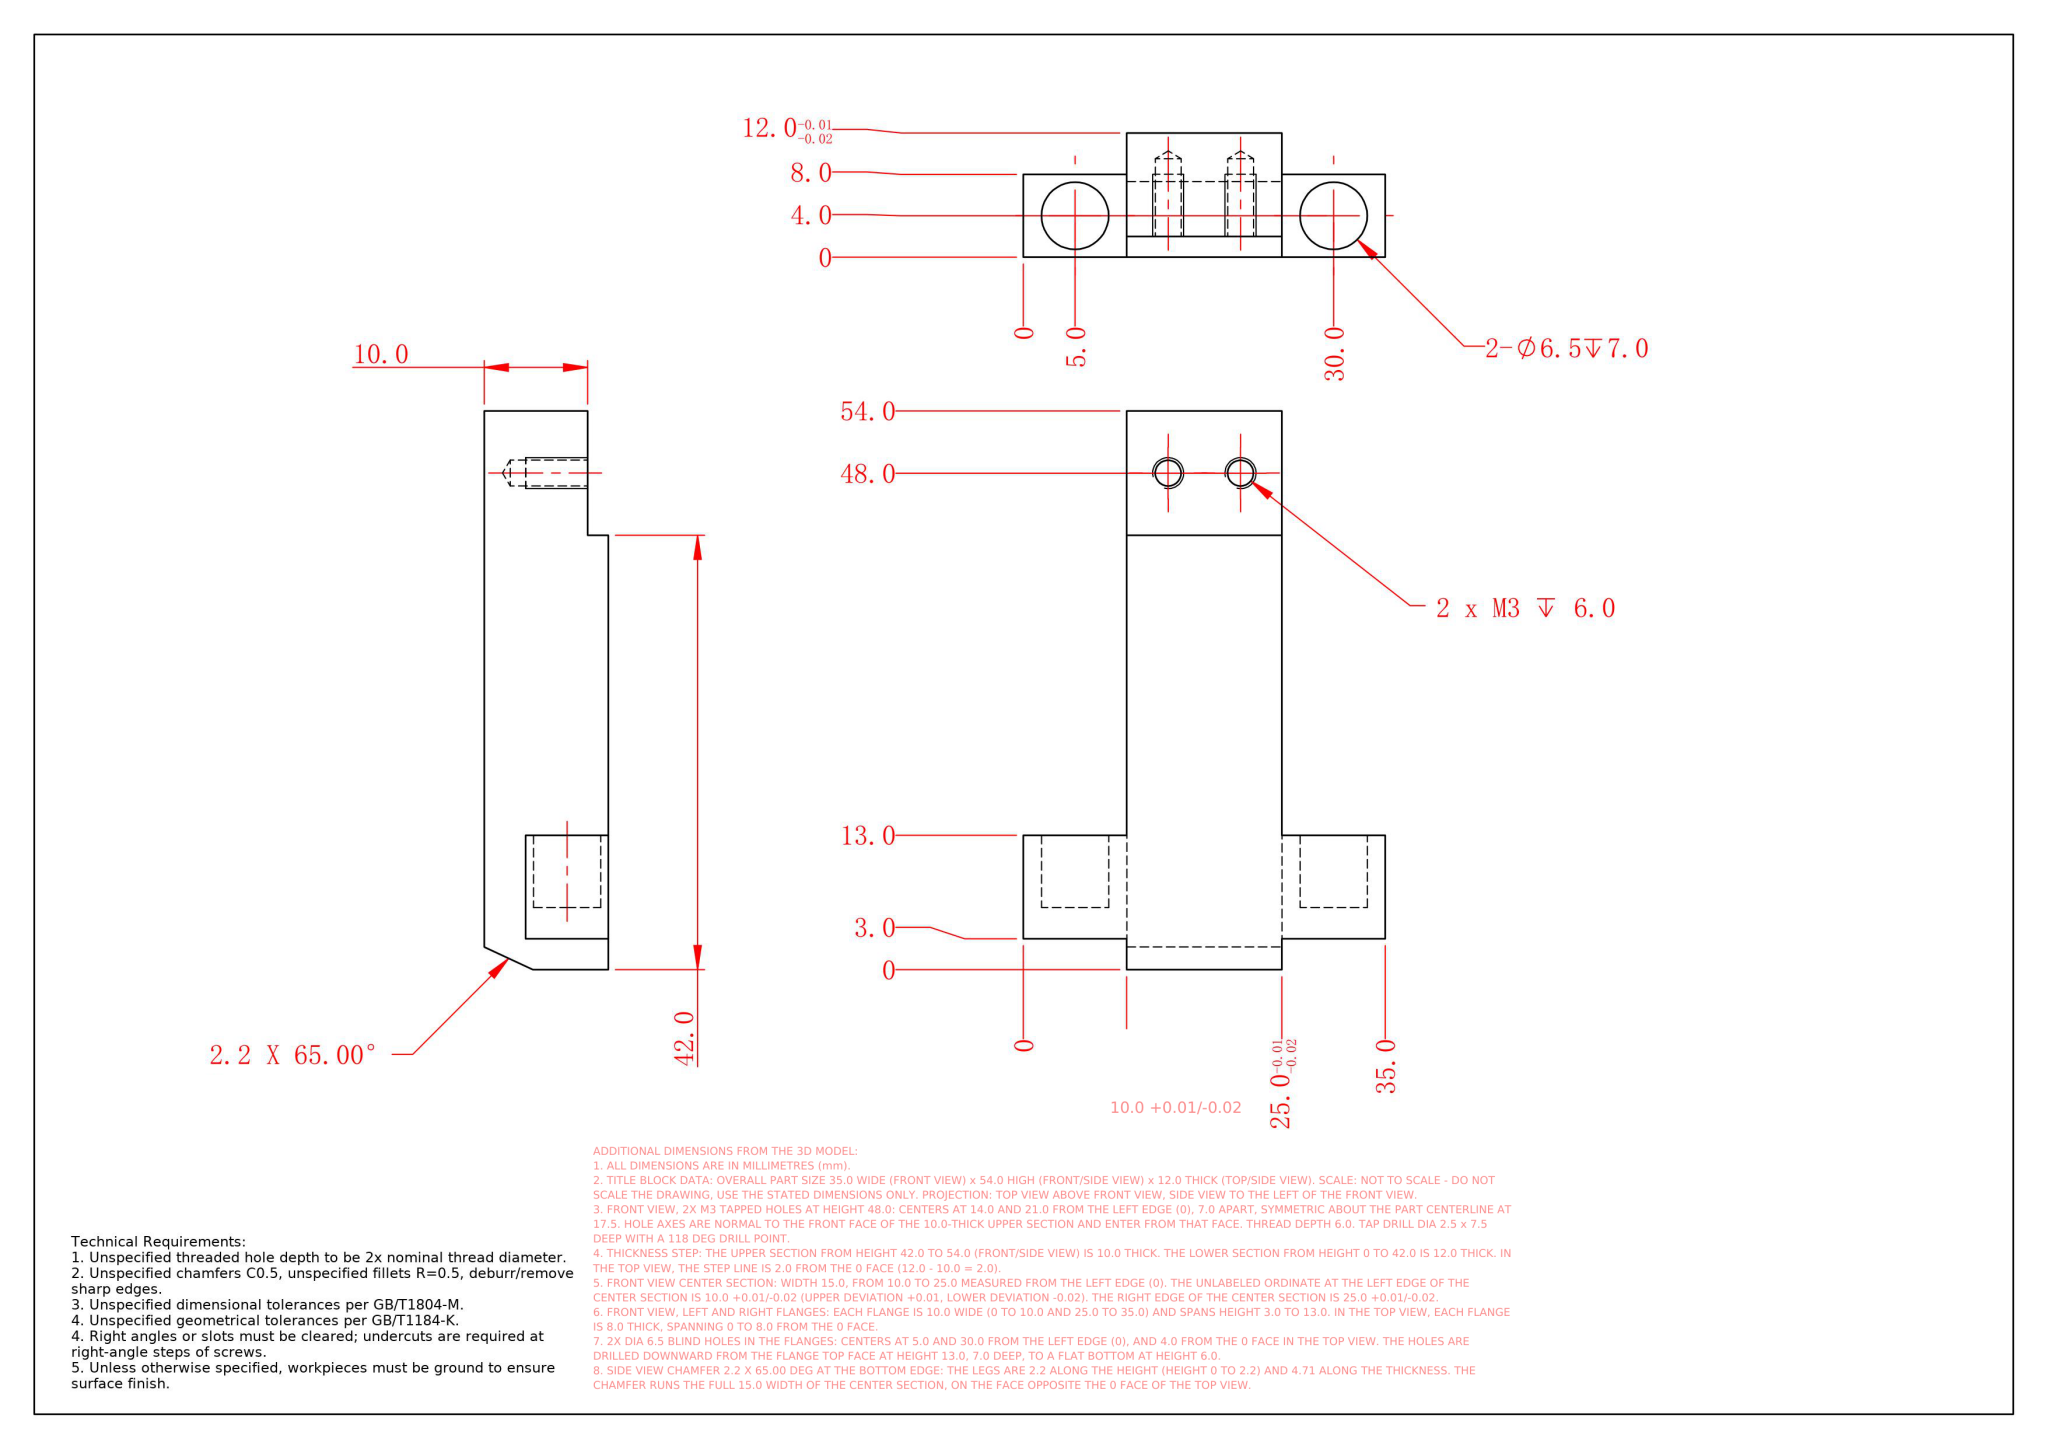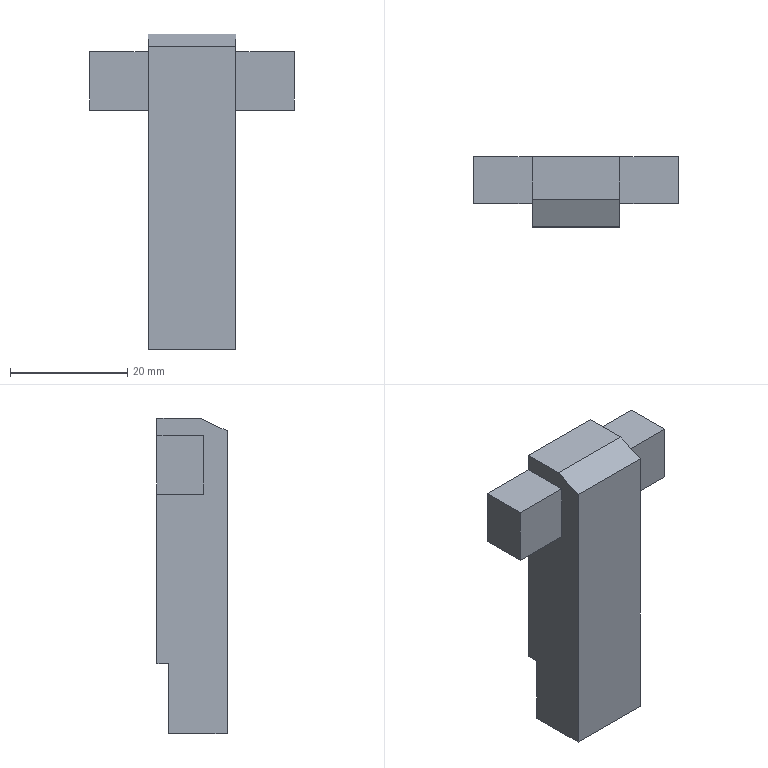Part | NX | mm | 1 solid | 31 faces | box 35 x 12 x 54 mm | volume 10342 mm3 | plane 19 | cylinder 8 | cone 4 | commonest cylinder face diameters 2.5 x4 6.5 x4
STEP:
#1=COLOUR_RGB('',0.7529,0.7529,0.7529);
#2=FILL_AREA_STYLE_COLOUR('',#1);
#3=FILL_AREA_STYLE('',(#2));
#4=SURFACE_STYLE_FILL_AREA(#3);
#5=SURFACE_SIDE_STYLE('',(#4));
#6=SURFACE_STYLE_USAGE(.BOTH.,#5);
#7=PRESENTATION_STYLE_ASSIGNMENT((#6));
#8=CARTESIAN_POINT('',(3.5,2.5,-23.25));
#9=VERTEX_POINT('',#8);
#10=CARTESIAN_POINT('',(3.5,2.5,-20.75));
#11=VERTEX_POINT('',#10);
#12=CARTESIAN_POINT('',(3.5,2.5,-22.));
#13=DIRECTION('',(0.,1.,0.));
#14=DIRECTION('',(0.,0.,1.));
#15=AXIS2_PLACEMENT_3D('',#12,#13,#14);
#16=CIRCLE('',#15,1.25);
#17=EDGE_CURVE('',#9,#11,#16,.T.);
#18=ORIENTED_EDGE('',*,*,#17,.F.);
#19=CARTESIAN_POINT('',(3.5,10.,-23.25));
#20=VERTEX_POINT('',#19);
#21=CARTESIAN_POINT('',(3.5,10.,-23.25));
#22=DIRECTION('',(0.,1.,0.));
#23=VECTOR('',#22,1000.);
#24=LINE('',#21,#23);
#25=EDGE_CURVE('',#9,#20,#24,.T.);
#26=ORIENTED_EDGE('',*,*,#25,.T.);
#27=CARTESIAN_POINT('',(3.5,10.,-20.75));
#28=VERTEX_POINT('',#27);
#29=CARTESIAN_POINT('',(3.5,10.,-22.));
#30=DIRECTION('',(0.,1.,0.));
#31=DIRECTION('',(0.,0.,1.));
#32=AXIS2_PLACEMENT_3D('',#29,#30,#31);
#33=CIRCLE('',#32,1.25);
#34=EDGE_CURVE('',#20,#28,#33,.T.);
#35=ORIENTED_EDGE('',*,*,#34,.T.);
#36=CARTESIAN_POINT('',(3.5,10.,-20.75));
#37=DIRECTION('',(0.,1.,0.));
#38=VECTOR('',#37,1000.);
#39=LINE('',#36,#38);
#40=EDGE_CURVE('',#11,#28,#39,.T.);
#41=ORIENTED_EDGE('',*,*,#40,.F.);
#42=EDGE_LOOP('',(#18,#26,#35,#41));
#43=FACE_OUTER_BOUND('',#42,.T.);
#44=CARTESIAN_POINT('',(3.5,10.,-22.));
#45=DIRECTION('',(0.,1.,0.));
#46=DIRECTION('',(0.,0.,1.));
#47=AXIS2_PLACEMENT_3D('',#44,#45,#46);
#48=CYLINDRICAL_SURFACE('',#47,1.25);
#49=ADVANCED_FACE('',(#43),#48,.F.);
#50=STYLED_ITEM('',(#7),#49);
#51=PRESENTATION_LAYER_ASSIGNMENT('','',(#50));
#52=COLOUR_RGB('',0.7529,0.7529,0.7529);
#53=FILL_AREA_STYLE_COLOUR('',#52);
#54=FILL_AREA_STYLE('',(#53));
#55=SURFACE_STYLE_FILL_AREA(#54);
#56=SURFACE_SIDE_STYLE('',(#55));
#57=SURFACE_STYLE_USAGE(.BOTH.,#56);
#58=PRESENTATION_STYLE_ASSIGNMENT((#57));
#59=ORIENTED_EDGE('',*,*,#25,.F.);
#60=CARTESIAN_POINT('',(3.5,2.5,-22.));
#61=DIRECTION('',(0.,1.,0.));
#62=DIRECTION('',(0.,0.,1.));
#63=AXIS2_PLACEMENT_3D('',#60,#61,#62);
#64=CIRCLE('',#63,1.25);
#65=EDGE_CURVE('',#11,#9,#64,.T.);
#66=ORIENTED_EDGE('',*,*,#65,.F.);
#67=ORIENTED_EDGE('',*,*,#40,.T.);
#68=CARTESIAN_POINT('',(3.5,10.,-22.));
#69=DIRECTION('',(0.,1.,0.));
#70=DIRECTION('',(0.,0.,1.));
#71=AXIS2_PLACEMENT_3D('',#68,#69,#70);
#72=CIRCLE('',#71,1.25);
#73=EDGE_CURVE('',#28,#20,#72,.T.);
#74=ORIENTED_EDGE('',*,*,#73,.T.);
#75=EDGE_LOOP('',(#59,#66,#67,#74));
#76=FACE_OUTER_BOUND('',#75,.T.);
#77=CARTESIAN_POINT('',(3.5,10.,-22.));
#78=DIRECTION('',(0.,1.,0.));
#79=DIRECTION('',(0.,0.,1.));
#80=AXIS2_PLACEMENT_3D('',#77,#78,#79);
#81=CYLINDRICAL_SURFACE('',#80,1.25);
#82=ADVANCED_FACE('',(#76),#81,.F.);
#83=STYLED_ITEM('',(#58),#82);
#84=PRESENTATION_LAYER_ASSIGNMENT('','',(#83));
#85=COLOUR_RGB('',0.7529,0.7529,0.7529);
#86=FILL_AREA_STYLE_COLOUR('',#85);
#87=FILL_AREA_STYLE('',(#86));
#88=SURFACE_STYLE_FILL_AREA(#87);
#89=SURFACE_SIDE_STYLE('',(#88));
#90=SURFACE_STYLE_USAGE(.BOTH.,#89);
#91=PRESENTATION_STYLE_ASSIGNMENT((#90));
#92=CARTESIAN_POINT('',(-3.5,2.5,-23.25));
#93=VERTEX_POINT('',#92);
#94=CARTESIAN_POINT('',(-3.5,2.5,-20.75));
#95=VERTEX_POINT('',#94);
#96=CARTESIAN_POINT('',(-3.5,2.5,-22.));
#97=DIRECTION('',(0.,1.,0.));
#98=DIRECTION('',(0.,0.,1.));
#99=AXIS2_PLACEMENT_3D('',#96,#97,#98);
#100=CIRCLE('',#99,1.25);
#101=EDGE_CURVE('',#93,#95,#100,.T.);
#102=ORIENTED_EDGE('',*,*,#101,.F.);
#103=CARTESIAN_POINT('',(-3.5,10.,-23.25));
#104=VERTEX_POINT('',#103);
#105=CARTESIAN_POINT('',(-3.5,10.,-23.25));
#106=DIRECTION('',(0.,1.,0.));
#107=VECTOR('',#106,1000.);
#108=LINE('',#105,#107);
#109=EDGE_CURVE('',#93,#104,#108,.T.);
#110=ORIENTED_EDGE('',*,*,#109,.T.);
#111=CARTESIAN_POINT('',(-3.5,10.,-20.75));
#112=VERTEX_POINT('',#111);
#113=CARTESIAN_POINT('',(-3.5,10.,-22.));
#114=DIRECTION('',(0.,1.,0.));
#115=DIRECTION('',(0.,0.,1.));
#116=AXIS2_PLACEMENT_3D('',#113,#114,#115);
#117=CIRCLE('',#116,1.25);
#118=EDGE_CURVE('',#104,#112,#117,.T.);
#119=ORIENTED_EDGE('',*,*,#118,.T.);
#120=CARTESIAN_POINT('',(-3.5,10.,-20.75));
#121=DIRECTION('',(0.,1.,0.));
#122=VECTOR('',#121,1000.);
#123=LINE('',#120,#122);
#124=EDGE_CURVE('',#95,#112,#123,.T.);
#125=ORIENTED_EDGE('',*,*,#124,.F.);
#126=EDGE_LOOP('',(#102,#110,#119,#125));
#127=FACE_OUTER_BOUND('',#126,.T.);
#128=CARTESIAN_POINT('',(-3.5,10.,-22.));
#129=DIRECTION('',(0.,1.,0.));
#130=DIRECTION('',(0.,0.,1.));
#131=AXIS2_PLACEMENT_3D('',#128,#129,#130);
#132=CYLINDRICAL_SURFACE('',#131,1.25);
#133=ADVANCED_FACE('',(#127),#132,.F.);
#134=STYLED_ITEM('',(#91),#133);
#135=PRESENTATION_LAYER_ASSIGNMENT('','',(#134));
#136=COLOUR_RGB('',0.7529,0.7529,0.7529);
#137=FILL_AREA_STYLE_COLOUR('',#136);
#138=FILL_AREA_STYLE('',(#137));
#139=SURFACE_STYLE_FILL_AREA(#138);
#140=SURFACE_SIDE_STYLE('',(#139));
#141=SURFACE_STYLE_USAGE(.BOTH.,#140);
#142=PRESENTATION_STYLE_ASSIGNMENT((#141));
#143=ORIENTED_EDGE('',*,*,#109,.F.);
#144=CARTESIAN_POINT('',(-3.5,2.5,-22.));
#145=DIRECTION('',(0.,1.,0.));
#146=DIRECTION('',(0.,0.,1.));
#147=AXIS2_PLACEMENT_3D('',#144,#145,#146);
#148=CIRCLE('',#147,1.25);
#149=EDGE_CURVE('',#95,#93,#148,.T.);
#150=ORIENTED_EDGE('',*,*,#149,.F.);
#151=ORIENTED_EDGE('',*,*,#124,.T.);
#152=CARTESIAN_POINT('',(-3.5,10.,-22.));
#153=DIRECTION('',(0.,1.,0.));
#154=DIRECTION('',(0.,0.,1.));
#155=AXIS2_PLACEMENT_3D('',#152,#153,#154);
#156=CIRCLE('',#155,1.25);
#157=EDGE_CURVE('',#112,#104,#156,.T.);
#158=ORIENTED_EDGE('',*,*,#157,.T.);
#159=EDGE_LOOP('',(#143,#150,#151,#158));
#160=FACE_OUTER_BOUND('',#159,.T.);
#161=CARTESIAN_POINT('',(-3.5,10.,-22.));
#162=DIRECTION('',(0.,1.,0.));
#163=DIRECTION('',(0.,0.,1.));
#164=AXIS2_PLACEMENT_3D('',#161,#162,#163);
#165=CYLINDRICAL_SURFACE('',#164,1.25);
#166=ADVANCED_FACE('',(#160),#165,.F.);
#167=STYLED_ITEM('',(#142),#166);
#168=(LENGTH_UNIT()NAMED_UNIT(*)SI_UNIT(.MILLI.,.METRE.));
#169=UNCERTAINTY_MEASURE_WITH_UNIT(LENGTH_MEASURE(0.00001),#168,'','');
#170=(NAMED_UNIT(*)PLANE_ANGLE_UNIT()SI_UNIT($,.RADIAN.));
#171=(NAMED_UNIT(*)SI_UNIT($,.STERADIAN.)SOLID_ANGLE_UNIT());
#172=(GEOMETRIC_REPRESENTATION_CONTEXT(3)GLOBAL_UNCERTAINTY_ASSIGNED_CONTEXT((#169))GLOBAL_UNIT_ASSIGNED_CONTEXT((#168,#170,#171))REPRESENTATION_CONTEXT('',''));
#173=MECHANICAL_DESIGN_GEOMETRIC_PRESENTATION_REPRESENTATION('',(#167),#172);
#174=COLOUR_RGB('',0.7529,0.7529,0.7529);
#175=FILL_AREA_STYLE_COLOUR('',#174);
#176=FILL_AREA_STYLE('',(#175));
#177=SURFACE_STYLE_FILL_AREA(#176);
#178=SURFACE_SIDE_STYLE('',(#177));
#179=SURFACE_STYLE_USAGE(.BOTH.,#178);
#180=PRESENTATION_STYLE_ASSIGNMENT((#179));
#181=CARTESIAN_POINT('',(3.5,1.749,-22.));
#182=VERTEX_POINT('',#181);
#183=CARTESIAN_POINT('',(3.5,2.5,-20.75));
#184=DIRECTION('',(0.,0.515,0.8572));
#185=VECTOR('',#184,1000.);
#186=LINE('',#183,#185);
#187=EDGE_CURVE('',#182,#11,#186,.T.);
#188=ORIENTED_EDGE('',*,*,#187,.F.);
#189=CARTESIAN_POINT('',(3.5,2.5,-23.25));
#190=DIRECTION('',(0.,0.515,-0.8572));
#191=VECTOR('',#190,1000.);
#192=LINE('',#189,#191);
#193=EDGE_CURVE('',#182,#9,#192,.T.);
#194=ORIENTED_EDGE('',*,*,#193,.T.);
#195=ORIENTED_EDGE('',*,*,#17,.T.);
#196=EDGE_LOOP('',(#188,#194,#195));
#197=FACE_OUTER_BOUND('',#196,.T.);
#198=CARTESIAN_POINT('',(3.5,2.5,-22.));
#199=DIRECTION('',(0.,1.,0.));
#200=DIRECTION('',(0.,0.,1.));
#201=AXIS2_PLACEMENT_3D('',#198,#199,#200);
#202=CONICAL_SURFACE('',#201,1.25,1.03);
#203=ADVANCED_FACE('',(#197),#202,.F.);
#204=CARTESIAN_POINT('',(-3.5,1.749,-22.));
#205=VERTEX_POINT('',#204);
#206=CARTESIAN_POINT('',(-3.5,2.5,-20.75));
#207=DIRECTION('',(0.,0.515,0.8572));
#208=VECTOR('',#207,1000.);
#209=LINE('',#206,#208);
#210=EDGE_CURVE('',#205,#95,#209,.T.);
#211=ORIENTED_EDGE('',*,*,#210,.F.);
#212=CARTESIAN_POINT('',(-3.5,2.5,-23.25));
#213=DIRECTION('',(0.,0.515,-0.8572));
#214=VECTOR('',#213,1000.);
#215=LINE('',#212,#214);
#216=EDGE_CURVE('',#205,#93,#215,.T.);
#217=ORIENTED_EDGE('',*,*,#216,.T.);
#218=ORIENTED_EDGE('',*,*,#101,.T.);
#219=EDGE_LOOP('',(#211,#217,#218));
#220=FACE_OUTER_BOUND('',#219,.T.);
#221=CARTESIAN_POINT('',(-3.5,2.5,-22.));
#222=DIRECTION('',(0.,1.,0.));
#223=DIRECTION('',(0.,0.,1.));
#224=AXIS2_PLACEMENT_3D('',#221,#222,#223);
#225=CONICAL_SURFACE('',#224,1.25,1.03);
#226=ADVANCED_FACE('',(#220),#225,.F.);
#227=CARTESIAN_POINT('',(15.75,8.,20.));
#228=VERTEX_POINT('',#227);
#229=CARTESIAN_POINT('',(9.25,8.,20.));
#230=VERTEX_POINT('',#229);
#231=CARTESIAN_POINT('',(12.5,8.,20.));
#232=DIRECTION('',(0.,0.,-1.));
#233=DIRECTION('',(-1.,0.,0.));
#234=AXIS2_PLACEMENT_3D('',#231,#232,#233);
#235=CIRCLE('',#234,3.25);
#236=EDGE_CURVE('',#228,#230,#235,.T.);
#237=ORIENTED_EDGE('',*,*,#236,.F.);
#238=CARTESIAN_POINT('',(15.75,8.,13.));
#239=VERTEX_POINT('',#238);
#240=CARTESIAN_POINT('',(15.75,8.,20.));
#241=DIRECTION('',(0.,0.,-1.));
#242=VECTOR('',#241,1000.);
#243=LINE('',#240,#242);
#244=EDGE_CURVE('',#228,#239,#243,.T.);
#245=ORIENTED_EDGE('',*,*,#244,.T.);
#246=CARTESIAN_POINT('',(9.25,8.,13.));
#247=VERTEX_POINT('',#246);
#248=CARTESIAN_POINT('',(12.5,8.,13.));
#249=DIRECTION('',(0.,0.,-1.));
#250=DIRECTION('',(-1.,0.,0.));
#251=AXIS2_PLACEMENT_3D('',#248,#249,#250);
#252=CIRCLE('',#251,3.25);
#253=EDGE_CURVE('',#239,#247,#252,.T.);
#254=ORIENTED_EDGE('',*,*,#253,.T.);
#255=CARTESIAN_POINT('',(9.25,8.,20.));
#256=DIRECTION('',(0.,0.,-1.));
#257=VECTOR('',#256,1000.);
#258=LINE('',#255,#257);
#259=EDGE_CURVE('',#230,#247,#258,.T.);
#260=ORIENTED_EDGE('',*,*,#259,.F.);
#261=EDGE_LOOP('',(#237,#245,#254,#260));
#262=FACE_OUTER_BOUND('',#261,.T.);
#263=CARTESIAN_POINT('',(12.5,8.,20.));
#264=DIRECTION('',(0.,0.,-1.));
#265=DIRECTION('',(-1.,0.,0.));
#266=AXIS2_PLACEMENT_3D('',#263,#264,#265);
#267=CYLINDRICAL_SURFACE('',#266,3.25);
#268=ADVANCED_FACE('',(#262),#267,.F.);
#269=CARTESIAN_POINT('',(-9.25,8.,20.));
#270=VERTEX_POINT('',#269);
#271=CARTESIAN_POINT('',(-15.75,8.,20.));
#272=VERTEX_POINT('',#271);
#273=CARTESIAN_POINT('',(-12.5,8.,20.));
#274=DIRECTION('',(0.,0.,-1.));
#275=DIRECTION('',(-1.,0.,0.));
#276=AXIS2_PLACEMENT_3D('',#273,#274,#275);
#277=CIRCLE('',#276,3.25);
#278=EDGE_CURVE('',#270,#272,#277,.T.);
#279=ORIENTED_EDGE('',*,*,#278,.F.);
#280=CARTESIAN_POINT('',(-9.25,8.,13.));
#281=VERTEX_POINT('',#280);
#282=CARTESIAN_POINT('',(-9.25,8.,20.));
#283=DIRECTION('',(0.,0.,-1.));
#284=VECTOR('',#283,1000.);
#285=LINE('',#282,#284);
#286=EDGE_CURVE('',#270,#281,#285,.T.);
#287=ORIENTED_EDGE('',*,*,#286,.T.);
#288=CARTESIAN_POINT('',(-15.75,8.,13.));
#289=VERTEX_POINT('',#288);
#290=CARTESIAN_POINT('',(-12.5,8.,13.));
#291=DIRECTION('',(0.,0.,-1.));
#292=DIRECTION('',(-1.,0.,0.));
#293=AXIS2_PLACEMENT_3D('',#290,#291,#292);
#294=CIRCLE('',#293,3.25);
#295=EDGE_CURVE('',#281,#289,#294,.T.);
#296=ORIENTED_EDGE('',*,*,#295,.T.);
#297=CARTESIAN_POINT('',(-15.75,8.,20.));
#298=DIRECTION('',(0.,0.,-1.));
#299=VECTOR('',#298,1000.);
#300=LINE('',#297,#299);
#301=EDGE_CURVE('',#272,#289,#300,.T.);
#302=ORIENTED_EDGE('',*,*,#301,.F.);
#303=EDGE_LOOP('',(#279,#287,#296,#302));
#304=FACE_OUTER_BOUND('',#303,.T.);
#305=CARTESIAN_POINT('',(-12.5,8.,20.));
#306=DIRECTION('',(0.,0.,-1.));
#307=DIRECTION('',(-1.,0.,0.));
#308=AXIS2_PLACEMENT_3D('',#305,#306,#307);
#309=CYLINDRICAL_SURFACE('',#308,3.25);
#310=ADVANCED_FACE('',(#304),#309,.F.);
#311=CARTESIAN_POINT('',(7.5,12.,26.));
#312=VERTEX_POINT('',#311);
#313=CARTESIAN_POINT('',(7.5,12.,23.));
#314=VERTEX_POINT('',#313);
#315=CARTESIAN_POINT('',(7.5,12.,-28.));
#316=DIRECTION('',(-0.,0.,-1.));
#317=VECTOR('',#316,1000.);
#318=LINE('',#315,#317);
#319=EDGE_CURVE('',#312,#314,#318,.T.);
#320=ORIENTED_EDGE('',*,*,#319,.F.);
#321=CARTESIAN_POINT('',(7.5,4.711,26.));
#322=VERTEX_POINT('',#321);
#323=CARTESIAN_POINT('',(7.5,-0.001,26.));
#324=DIRECTION('',(0.,1.,0.));
#325=VECTOR('',#324,1000.);
#326=LINE('',#323,#325);
#327=EDGE_CURVE('',#322,#312,#326,.T.);
#328=ORIENTED_EDGE('',*,*,#327,.F.);
#329=CARTESIAN_POINT('',(7.5,-0.,23.803));
#330=VERTEX_POINT('',#329);
#331=CARTESIAN_POINT('',(7.5,9.,28.));
#332=DIRECTION('',(0.,0.9063,0.4226));
#333=VECTOR('',#332,1000.);
#334=LINE('',#331,#333);
#335=EDGE_CURVE('',#330,#322,#334,.T.);
#336=ORIENTED_EDGE('',*,*,#335,.F.);
#337=CARTESIAN_POINT('',(7.5,0.,-28.));
#338=VERTEX_POINT('',#337);
#339=CARTESIAN_POINT('',(7.5,0.,-28.));
#340=DIRECTION('',(-0.,0.,-1.));
#341=VECTOR('',#340,1000.);
#342=LINE('',#339,#341);
#343=EDGE_CURVE('',#330,#338,#342,.T.);
#344=ORIENTED_EDGE('',*,*,#343,.T.);
#345=CARTESIAN_POINT('',(7.5,10.,-28.));
#346=VERTEX_POINT('',#345);
#347=CARTESIAN_POINT('',(7.5,12.,-28.));
#348=DIRECTION('',(0.,-1.,0.));
#349=VECTOR('',#348,1000.);
#350=LINE('',#347,#349);
#351=EDGE_CURVE('',#346,#338,#350,.T.);
#352=ORIENTED_EDGE('',*,*,#351,.F.);
#353=CARTESIAN_POINT('',(7.5,10.,-16.));
#354=VERTEX_POINT('',#353);
#355=CARTESIAN_POINT('',(7.5,10.,-28.));
#356=DIRECTION('',(0.,0.,1.));
#357=VECTOR('',#356,1000.);
#358=LINE('',#355,#357);
#359=EDGE_CURVE('',#346,#354,#358,.T.);
#360=ORIENTED_EDGE('',*,*,#359,.T.);
#361=CARTESIAN_POINT('',(7.5,12.,-16.));
#362=VERTEX_POINT('',#361);
#363=CARTESIAN_POINT('',(7.5,12.,-16.));
#364=DIRECTION('',(0.,1.,0.));
#365=VECTOR('',#364,1000.);
#366=LINE('',#363,#365);
#367=EDGE_CURVE('',#354,#362,#366,.T.);
#368=ORIENTED_EDGE('',*,*,#367,.T.);
#369=CARTESIAN_POINT('',(7.5,12.,13.));
#370=VERTEX_POINT('',#369);
#371=CARTESIAN_POINT('',(7.5,12.,-28.));
#372=DIRECTION('',(-0.,0.,-1.));
#373=VECTOR('',#372,1000.);
#374=LINE('',#371,#373);
#375=EDGE_CURVE('',#370,#362,#374,.T.);
#376=ORIENTED_EDGE('',*,*,#375,.F.);
#377=CARTESIAN_POINT('',(7.5,4.,13.));
#378=VERTEX_POINT('',#377);
#379=CARTESIAN_POINT('',(7.5,4.,13.));
#380=DIRECTION('',(0.,1.,0.));
#381=VECTOR('',#380,1000.);
#382=LINE('',#379,#381);
#383=EDGE_CURVE('',#378,#370,#382,.T.);
#384=ORIENTED_EDGE('',*,*,#383,.F.);
#385=CARTESIAN_POINT('',(7.5,4.,23.));
#386=VERTEX_POINT('',#385);
#387=CARTESIAN_POINT('',(7.5,4.,23.));
#388=DIRECTION('',(0.,0.,1.));
#389=VECTOR('',#388,1000.);
#390=LINE('',#387,#389);
#391=EDGE_CURVE('',#378,#386,#390,.T.);
#392=ORIENTED_EDGE('',*,*,#391,.T.);
#393=CARTESIAN_POINT('',(7.5,4.,23.));
#394=DIRECTION('',(0.,1.,0.));
#395=VECTOR('',#394,1000.);
#396=LINE('',#393,#395);
#397=EDGE_CURVE('',#386,#314,#396,.T.);
#398=ORIENTED_EDGE('',*,*,#397,.T.);
#399=EDGE_LOOP('',(#320,#328,#336,#344,#352,#360,#368,#376,#384,#392,#398));
#400=FACE_OUTER_BOUND('',#399,.T.);
#401=CARTESIAN_POINT('',(7.5,12.,-28.));
#402=DIRECTION('',(-1.,0.,0.));
#403=DIRECTION('',(0.,0.,1.));
#404=AXIS2_PLACEMENT_3D('',#401,#402,#403);
#405=PLANE('',#404);
#406=ADVANCED_FACE('',(#400),#405,.F.);
#407=CARTESIAN_POINT('',(-7.5,0.,23.803));
#408=VERTEX_POINT('',#407);
#409=CARTESIAN_POINT('',(-7.5,4.711,26.));
#410=VERTEX_POINT('',#409);
#411=CARTESIAN_POINT('',(-7.5,9.,28.));
#412=DIRECTION('',(0.,0.9063,0.4226));
#413=VECTOR('',#412,1000.);
#414=LINE('',#411,#413);
#415=EDGE_CURVE('',#408,#410,#414,.T.);
#416=ORIENTED_EDGE('',*,*,#415,.T.);
#417=CARTESIAN_POINT('',(-7.5,12.,26.));
#418=VERTEX_POINT('',#417);
#419=CARTESIAN_POINT('',(-7.5,-0.001,26.));
#420=DIRECTION('',(0.,1.,0.));
#421=VECTOR('',#420,1000.);
#422=LINE('',#419,#421);
#423=EDGE_CURVE('',#410,#418,#422,.T.);
#424=ORIENTED_EDGE('',*,*,#423,.T.);
#425=CARTESIAN_POINT('',(-7.5,12.,23.));
#426=VERTEX_POINT('',#425);
#427=CARTESIAN_POINT('',(-7.5,12.,-28.));
#428=DIRECTION('',(0.,0.,1.));
#429=VECTOR('',#428,1000.);
#430=LINE('',#427,#429);
#431=EDGE_CURVE('',#426,#418,#430,.T.);
#432=ORIENTED_EDGE('',*,*,#431,.F.);
#433=CARTESIAN_POINT('',(-7.5,4.,23.));
#434=VERTEX_POINT('',#433);
#435=CARTESIAN_POINT('',(-7.5,4.,23.));
#436=DIRECTION('',(0.,1.,0.));
#437=VECTOR('',#436,1000.);
#438=LINE('',#435,#437);
#439=EDGE_CURVE('',#434,#426,#438,.T.);
#440=ORIENTED_EDGE('',*,*,#439,.F.);
#441=CARTESIAN_POINT('',(-7.5,4.,13.));
#442=VERTEX_POINT('',#441);
#443=CARTESIAN_POINT('',(-7.5,4.,23.));
#444=DIRECTION('',(0.,0.,-1.));
#445=VECTOR('',#444,1000.);
#446=LINE('',#443,#445);
#447=EDGE_CURVE('',#434,#442,#446,.T.);
#448=ORIENTED_EDGE('',*,*,#447,.T.);
#449=CARTESIAN_POINT('',(-7.5,12.,13.));
#450=VERTEX_POINT('',#449);
#451=CARTESIAN_POINT('',(-7.5,4.,13.));
#452=DIRECTION('',(0.,1.,0.));
#453=VECTOR('',#452,1000.);
#454=LINE('',#451,#453);
#455=EDGE_CURVE('',#442,#450,#454,.T.);
#456=ORIENTED_EDGE('',*,*,#455,.T.);
#457=CARTESIAN_POINT('',(-7.5,12.,-16.));
#458=VERTEX_POINT('',#457);
#459=CARTESIAN_POINT('',(-7.5,12.,-28.));
#460=DIRECTION('',(0.,0.,1.));
#461=VECTOR('',#460,1000.);
#462=LINE('',#459,#461);
#463=EDGE_CURVE('',#458,#450,#462,.T.);
#464=ORIENTED_EDGE('',*,*,#463,.F.);
#465=CARTESIAN_POINT('',(-7.5,10.,-16.));
#466=VERTEX_POINT('',#465);
#467=CARTESIAN_POINT('',(-7.5,12.,-16.));
#468=DIRECTION('',(0.,1.,0.));
#469=VECTOR('',#468,1000.);
#470=LINE('',#467,#469);
#471=EDGE_CURVE('',#466,#458,#470,.T.);
#472=ORIENTED_EDGE('',*,*,#471,.F.);
#473=CARTESIAN_POINT('',(-7.5,10.,-28.));
#474=VERTEX_POINT('',#473);
#475=CARTESIAN_POINT('',(-7.5,10.,-28.));
#476=DIRECTION('',(0.,0.,1.));
#477=VECTOR('',#476,1000.);
#478=LINE('',#475,#477);
#479=EDGE_CURVE('',#474,#466,#478,.T.);
#480=ORIENTED_EDGE('',*,*,#479,.F.);
#481=CARTESIAN_POINT('',(-7.5,0.,-28.));
#482=VERTEX_POINT('',#481);
#483=CARTESIAN_POINT('',(-7.5,12.,-28.));
#484=DIRECTION('',(0.,-1.,0.));
#485=VECTOR('',#484,1000.);
#486=LINE('',#483,#485);
#487=EDGE_CURVE('',#474,#482,#486,.T.);
#488=ORIENTED_EDGE('',*,*,#487,.T.);
#489=CARTESIAN_POINT('',(-7.5,0.,-28.));
#490=DIRECTION('',(0.,0.,1.));
#491=VECTOR('',#490,1000.);
#492=LINE('',#489,#491);
#493=EDGE_CURVE('',#482,#408,#492,.T.);
#494=ORIENTED_EDGE('',*,*,#493,.T.);
#495=EDGE_LOOP('',(#416,#424,#432,#440,#448,#456,#464,#472,#480,#488,#494));
#496=FACE_OUTER_BOUND('',#495,.T.);
#497=CARTESIAN_POINT('',(-7.5,12.,-28.));
#498=DIRECTION('',(1.,0.,-0.));
#499=DIRECTION('',(-0.,0.,-1.));
#500=AXIS2_PLACEMENT_3D('',#497,#498,#499);
#501=PLANE('',#500);
#502=ADVANCED_FACE('',(#496),#501,.F.);
#503=ORIENTED_EDGE('',*,*,#487,.F.);
#504=CARTESIAN_POINT('',(17.5,10.,-28.));
#505=DIRECTION('',(-1.,0.,0.));
#506=VECTOR('',#505,1000.);
#507=LINE('',#504,#506);
#508=EDGE_CURVE('',#346,#474,#507,.T.);
#509=ORIENTED_EDGE('',*,*,#508,.F.);
#510=ORIENTED_EDGE('',*,*,#351,.T.);
#511=CARTESIAN_POINT('',(-7.5,0.,-28.));
#512=DIRECTION('',(-1.,0.,0.));
#513=VECTOR('',#512,1000.);
#514=LINE('',#511,#513);
#515=EDGE_CURVE('',#338,#482,#514,.T.);
#516=ORIENTED_EDGE('',*,*,#515,.T.);
#517=EDGE_LOOP('',(#503,#509,#510,#516));
#518=FACE_OUTER_BOUND('',#517,.T.);
#519=CARTESIAN_POINT('',(-7.5,12.,-28.));
#520=DIRECTION('',(0.,0.,1.));
#521=DIRECTION('',(1.,0.,0.));
#522=AXIS2_PLACEMENT_3D('',#519,#520,#521);
#523=PLANE('',#522);
#524=ADVANCED_FACE('',(#518),#523,.F.);
#525=CARTESIAN_POINT('',(-7.5,12.,26.));
#526=DIRECTION('',(-1.,0.,0.));
#527=VECTOR('',#526,1000.);
#528=LINE('',#525,#527);
#529=EDGE_CURVE('',#312,#418,#528,.T.);
#530=ORIENTED_EDGE('',*,*,#529,.F.);
#531=ORIENTED_EDGE('',*,*,#319,.T.);
#532=CARTESIAN_POINT('',(17.5,12.,23.));
#533=VERTEX_POINT('',#532);
#534=CARTESIAN_POINT('',(7.5,12.,23.));
#535=DIRECTION('',(1.,0.,0.));
#536=VECTOR('',#535,1000.);
#537=LINE('',#534,#536);
#538=EDGE_CURVE('',#314,#533,#537,.T.);
#539=ORIENTED_EDGE('',*,*,#538,.T.);
#540=CARTESIAN_POINT('',(17.5,12.,13.));
#541=VERTEX_POINT('',#540);
#542=CARTESIAN_POINT('',(17.5,12.,23.));
#543=DIRECTION('',(0.,0.,-1.));
#544=VECTOR('',#543,1000.);
#545=LINE('',#542,#544);
#546=EDGE_CURVE('',#533,#541,#545,.T.);
#547=ORIENTED_EDGE('',*,*,#546,.T.);
#548=CARTESIAN_POINT('',(7.5,12.,13.));
#549=DIRECTION('',(-1.,0.,0.));
#550=VECTOR('',#549,1000.);
#551=LINE('',#548,#550);
#552=EDGE_CURVE('',#541,#370,#551,.T.);
#553=ORIENTED_EDGE('',*,*,#552,.T.);
#554=ORIENTED_EDGE('',*,*,#375,.T.);
#555=CARTESIAN_POINT('',(-0.,12.,-16.));
#556=DIRECTION('',(1.,0.,-0.));
#557=VECTOR('',#556,1000.);
#558=LINE('',#555,#557);
#559=EDGE_CURVE('',#458,#362,#558,.T.);
#560=ORIENTED_EDGE('',*,*,#559,.F.);
#561=ORIENTED_EDGE('',*,*,#463,.T.);
#562=CARTESIAN_POINT('',(-17.5,12.,13.));
#563=VERTEX_POINT('',#562);
#564=CARTESIAN_POINT('',(-7.5,12.,13.));
#565=DIRECTION('',(-1.,0.,0.));
#566=VECTOR('',#565,1000.);
#567=LINE('',#564,#566);
#568=EDGE_CURVE('',#450,#563,#567,.T.);
#569=ORIENTED_EDGE('',*,*,#568,.T.);
#570=CARTESIAN_POINT('',(-17.5,12.,23.));
#571=VERTEX_POINT('',#570);
#572=CARTESIAN_POINT('',(-17.5,12.,23.));
#573=DIRECTION('',(0.,0.,1.));
#574=VECTOR('',#573,1000.);
#575=LINE('',#572,#574);
#576=EDGE_CURVE('',#563,#571,#575,.T.);
#577=ORIENTED_EDGE('',*,*,#576,.T.);
#578=CARTESIAN_POINT('',(-7.5,12.,23.));
#579=DIRECTION('',(1.,0.,0.));
#580=VECTOR('',#579,1000.);
#581=LINE('',#578,#580);
#582=EDGE_CURVE('',#571,#426,#581,.T.);
#583=ORIENTED_EDGE('',*,*,#582,.T.);
#584=ORIENTED_EDGE('',*,*,#431,.T.);
#585=EDGE_LOOP('',(#530,#531,#539,#547,#553,#554,#560,#561,#569,#577,#583,#584));
#586=FACE_OUTER_BOUND('',#585,.T.);
#587=CARTESIAN_POINT('',(0.,12.,0.));
#588=DIRECTION('',(0.,1.,0.));
#589=DIRECTION('',(0.,0.,1.));
#590=AXIS2_PLACEMENT_3D('',#587,#588,#589);
#591=PLANE('',#590);
#592=ADVANCED_FACE('',(#586),#591,.T.);
#593=ORIENTED_EDGE('',*,*,#343,.F.);
#594=CARTESIAN_POINT('',(-7.5,-0.,23.803));
#595=DIRECTION('',(1.,0.,-0.));
#596=VECTOR('',#595,1000.);
#597=LINE('',#594,#596);
#598=EDGE_CURVE('',#408,#330,#597,.T.);
#599=ORIENTED_EDGE('',*,*,#598,.F.);
#600=ORIENTED_EDGE('',*,*,#493,.F.);
#601=ORIENTED_EDGE('',*,*,#515,.F.);
#602=EDGE_LOOP('',(#593,#599,#600,#601));
#603=FACE_OUTER_BOUND('',#602,.T.);
#604=CARTESIAN_POINT('',(0.,0.,0.));
#605=DIRECTION('',(0.,1.,0.));
#606=DIRECTION('',(0.,0.,1.));
#607=AXIS2_PLACEMENT_3D('',#604,#605,#606);
#608=PLANE('',#607);
#609=ADVANCED_FACE('',(#603),#608,.F.);
#610=ORIENTED_EDGE('',*,*,#335,.T.);
#611=CARTESIAN_POINT('',(-7.5,4.711,26.));
#612=DIRECTION('',(1.,0.,0.));
#613=VECTOR('',#612,1000.);
#614=LINE('',#611,#613);
#615=EDGE_CURVE('',#410,#322,#614,.T.);
#616=ORIENTED_EDGE('',*,*,#615,.F.);
#617=ORIENTED_EDGE('',*,*,#415,.F.);
#618=ORIENTED_EDGE('',*,*,#598,.T.);
#619=EDGE_LOOP('',(#610,#616,#617,#618));
#620=FACE_OUTER_BOUND('',#619,.T.);
#621=CARTESIAN_POINT('',(-7.5,9.,28.));
#622=DIRECTION('',(-0.,0.4226,-0.9063));
#623=DIRECTION('',(0.,0.9063,0.4226));
#624=AXIS2_PLACEMENT_3D('',#621,#622,#623);
#625=PLANE('',#624);
#626=ADVANCED_FACE('',(#620),#625,.F.);
#627=ORIENTED_EDGE('',*,*,#582,.F.);
#628=CARTESIAN_POINT('',(-17.5,4.,23.));
#629=VERTEX_POINT('',#628);
#630=CARTESIAN_POINT('',(-17.5,4.,23.));
#631=DIRECTION('',(0.,1.,0.));
#632=VECTOR('',#631,1000.);
#633=LINE('',#630,#632);
#634=EDGE_CURVE('',#629,#571,#633,.T.);
#635=ORIENTED_EDGE('',*,*,#634,.F.);
#636=CARTESIAN_POINT('',(-7.5,4.,23.));
#637=DIRECTION('',(1.,0.,0.));
#638=VECTOR('',#637,1000.);
#639=LINE('',#636,#638);
#640=EDGE_CURVE('',#629,#434,#639,.T.);
#641=ORIENTED_EDGE('',*,*,#640,.T.);
#642=ORIENTED_EDGE('',*,*,#439,.T.);
#643=EDGE_LOOP('',(#627,#635,#641,#642));
#644=FACE_OUTER_BOUND('',#643,.T.);
#645=CARTESIAN_POINT('',(-7.5,4.,23.));
#646=DIRECTION('',(-0.,0.,1.));
#647=DIRECTION('',(1.,0.,0.));
#648=AXIS2_PLACEMENT_3D('',#645,#646,#647);
#649=PLANE('',#648);
#650=ADVANCED_FACE('',(#644),#649,.T.);
#651=ORIENTED_EDGE('',*,*,#576,.F.);
#652=CARTESIAN_POINT('',(-17.5,4.,13.));
#653=VERTEX_POINT('',#652);
#654=CARTESIAN_POINT('',(-17.5,4.,13.));
#655=DIRECTION('',(0.,1.,0.));
#656=VECTOR('',#655,1000.);
#657=LINE('',#654,#656);
#658=EDGE_CURVE('',#653,#563,#657,.T.);
#659=ORIENTED_EDGE('',*,*,#658,.F.);
#660=CARTESIAN_POINT('',(-17.5,4.,23.));
#661=DIRECTION('',(0.,0.,1.));
#662=VECTOR('',#661,1000.);
#663=LINE('',#660,#662);
#664=EDGE_CURVE('',#653,#629,#663,.T.);
#665=ORIENTED_EDGE('',*,*,#664,.T.);
#666=ORIENTED_EDGE('',*,*,#634,.T.);
#667=EDGE_LOOP('',(#651,#659,#665,#666));
#668=FACE_OUTER_BOUND('',#667,.T.);
#669=CARTESIAN_POINT('',(-17.5,4.,23.));
#670=DIRECTION('',(-1.,0.,0.));
#671=DIRECTION('',(0.,0.,1.));
#672=AXIS2_PLACEMENT_3D('',#669,#670,#671);
#673=PLANE('',#672);
#674=ADVANCED_FACE('',(#668),#673,.T.);
#675=CARTESIAN_POINT('',(-12.5,8.,13.));
#676=DIRECTION('',(0.,0.,-1.));
#677=DIRECTION('',(-1.,0.,0.));
#678=AXIS2_PLACEMENT_3D('',#675,#676,#677);
#679=CIRCLE('',#678,3.25);
#680=EDGE_CURVE('',#289,#281,#679,.T.);
#681=ORIENTED_EDGE('',*,*,#680,.F.);
#682=ORIENTED_EDGE('',*,*,#295,.F.);
#683=EDGE_LOOP('',(#681,#682));
#684=FACE_BOUND('',#683,.T.);
#685=ORIENTED_EDGE('',*,*,#568,.F.);
#686=ORIENTED_EDGE('',*,*,#455,.F.);
#687=CARTESIAN_POINT('',(-7.5,4.,13.));
#688=DIRECTION('',(-1.,0.,0.));
#689=VECTOR('',#688,1000.);
#690=LINE('',#687,#689);
#691=EDGE_CURVE('',#442,#653,#690,.T.);
#692=ORIENTED_EDGE('',*,*,#691,.T.);
#693=ORIENTED_EDGE('',*,*,#658,.T.);
#694=EDGE_LOOP('',(#685,#686,#692,#693));
#695=FACE_OUTER_BOUND('',#694,.T.);
#696=CARTESIAN_POINT('',(-7.5,4.,13.));
#697=DIRECTION('',(-0.,0.,-1.));
#698=DIRECTION('',(-1.,0.,0.));
#699=AXIS2_PLACEMENT_3D('',#696,#697,#698);
#700=PLANE('',#699);
#701=ADVANCED_FACE('',(#684,#695),#700,.T.);
#702=ORIENTED_EDGE('',*,*,#447,.F.);
#703=ORIENTED_EDGE('',*,*,#640,.F.);
#704=ORIENTED_EDGE('',*,*,#664,.F.);
#705=ORIENTED_EDGE('',*,*,#691,.F.);
#706=EDGE_LOOP('',(#702,#703,#704,#705));
#707=FACE_OUTER_BOUND('',#706,.T.);
#708=CARTESIAN_POINT('',(0.,4.,0.));
#709=DIRECTION('',(0.,1.,0.));
#710=DIRECTION('',(0.,0.,1.));
#711=AXIS2_PLACEMENT_3D('',#708,#709,#710);
#712=PLANE('',#711);
#713=ADVANCED_FACE('',(#707),#712,.F.);
#714=CARTESIAN_POINT('',(12.5,8.,13.));
#715=DIRECTION('',(0.,0.,-1.));
#716=DIRECTION('',(-1.,0.,0.));
#717=AXIS2_PLACEMENT_3D('',#714,#715,#716);
#718=CIRCLE('',#717,3.25);
#719=EDGE_CURVE('',#247,#239,#718,.T.);
#720=ORIENTED_EDGE('',*,*,#719,.F.);
#721=ORIENTED_EDGE('',*,*,#253,.F.);
#722=EDGE_LOOP('',(#720,#721));
#723=FACE_BOUND('',#722,.T.);
#724=ORIENTED_EDGE('',*,*,#552,.F.);
#725=CARTESIAN_POINT('',(17.5,4.,13.));
#726=VERTEX_POINT('',#725);
#727=CARTESIAN_POINT('',(17.5,4.,13.));
#728=DIRECTION('',(0.,1.,0.));
#729=VECTOR('',#728,1000.);
#730=LINE('',#727,#729);
#731=EDGE_CURVE('',#726,#541,#730,.T.);
#732=ORIENTED_EDGE('',*,*,#731,.F.);
#733=CARTESIAN_POINT('',(7.5,4.,13.));
#734=DIRECTION('',(-1.,0.,0.));
#735=VECTOR('',#734,1000.);
#736=LINE('',#733,#735);
#737=EDGE_CURVE('',#726,#378,#736,.T.);
#738=ORIENTED_EDGE('',*,*,#737,.T.);
#739=ORIENTED_EDGE('',*,*,#383,.T.);
#740=EDGE_LOOP('',(#724,#732,#738,#739));
#741=FACE_OUTER_BOUND('',#740,.T.);
#742=CARTESIAN_POINT('',(7.5,4.,13.));
#743=DIRECTION('',(0.,0.,-1.));
#744=DIRECTION('',(-1.,0.,0.));
#745=AXIS2_PLACEMENT_3D('',#742,#743,#744);
#746=PLANE('',#745);
#747=ADVANCED_FACE('',(#723,#741),#746,.T.);
#748=ORIENTED_EDGE('',*,*,#546,.F.);
#749=CARTESIAN_POINT('',(17.5,4.,23.));
#750=VERTEX_POINT('',#749);
#751=CARTESIAN_POINT('',(17.5,4.,23.));
#752=DIRECTION('',(0.,1.,0.));
#753=VECTOR('',#752,1000.);
#754=LINE('',#751,#753);
#755=EDGE_CURVE('',#750,#533,#754,.T.);
#756=ORIENTED_EDGE('',*,*,#755,.F.);
#757=CARTESIAN_POINT('',(17.5,4.,23.));
#758=DIRECTION('',(0.,0.,-1.));
#759=VECTOR('',#758,1000.);
#760=LINE('',#757,#759);
#761=EDGE_CURVE('',#750,#726,#760,.T.);
#762=ORIENTED_EDGE('',*,*,#761,.T.);
#763=ORIENTED_EDGE('',*,*,#731,.T.);
#764=EDGE_LOOP('',(#748,#756,#762,#763));
#765=FACE_OUTER_BOUND('',#764,.T.);
#766=CARTESIAN_POINT('',(17.5,4.,23.));
#767=DIRECTION('',(1.,0.,0.));
#768=DIRECTION('',(0.,0.,-1.));
#769=AXIS2_PLACEMENT_3D('',#766,#767,#768);
#770=PLANE('',#769);
#771=ADVANCED_FACE('',(#765),#770,.T.);
#772=ORIENTED_EDGE('',*,*,#538,.F.);
#773=ORIENTED_EDGE('',*,*,#397,.F.);
#774=CARTESIAN_POINT('',(7.5,4.,23.));
#775=DIRECTION('',(1.,0.,0.));
#776=VECTOR('',#775,1000.);
#777=LINE('',#774,#776);
#778=EDGE_CURVE('',#386,#750,#777,.T.);
#779=ORIENTED_EDGE('',*,*,#778,.T.);
#780=ORIENTED_EDGE('',*,*,#755,.T.);
#781=EDGE_LOOP('',(#772,#773,#779,#780));
#782=FACE_OUTER_BOUND('',#781,.T.);
#783=CARTESIAN_POINT('',(7.5,4.,23.));
#784=DIRECTION('',(0.,0.,1.));
#785=DIRECTION('',(1.,0.,0.));
#786=AXIS2_PLACEMENT_3D('',#783,#784,#785);
#787=PLANE('',#786);
#788=ADVANCED_FACE('',(#782),#787,.T.);
#789=ORIENTED_EDGE('',*,*,#391,.F.);
#790=ORIENTED_EDGE('',*,*,#737,.F.);
#791=ORIENTED_EDGE('',*,*,#761,.F.);
#792=ORIENTED_EDGE('',*,*,#778,.F.);
#793=EDGE_LOOP('',(#789,#790,#791,#792));
#794=FACE_OUTER_BOUND('',#793,.T.);
#795=CARTESIAN_POINT('',(0.,4.,0.));
#796=DIRECTION('',(0.,-1.,0.));
#797=DIRECTION('',(0.,0.,-1.));
#798=AXIS2_PLACEMENT_3D('',#795,#796,#797);
#799=PLANE('',#798);
#800=ADVANCED_FACE('',(#794),#799,.T.);
#801=ORIENTED_EDGE('',*,*,#286,.F.);
#802=CARTESIAN_POINT('',(-12.5,8.,20.));
#803=DIRECTION('',(0.,0.,-1.));
#804=DIRECTION('',(-1.,0.,0.));
#805=AXIS2_PLACEMENT_3D('',#802,#803,#804);
#806=CIRCLE('',#805,3.25);
#807=EDGE_CURVE('',#272,#270,#806,.T.);
#808=ORIENTED_EDGE('',*,*,#807,.F.);
#809=ORIENTED_EDGE('',*,*,#301,.T.);
#810=ORIENTED_EDGE('',*,*,#680,.T.);
#811=EDGE_LOOP('',(#801,#808,#809,#810));
#812=FACE_OUTER_BOUND('',#811,.T.);
#813=CARTESIAN_POINT('',(-12.5,8.,20.));
#814=DIRECTION('',(0.,0.,-1.));
#815=DIRECTION('',(-1.,0.,0.));
#816=AXIS2_PLACEMENT_3D('',#813,#814,#815);
#817=CYLINDRICAL_SURFACE('',#816,3.25);
#818=ADVANCED_FACE('',(#812),#817,.F.);
#819=ORIENTED_EDGE('',*,*,#807,.T.);
#820=ORIENTED_EDGE('',*,*,#278,.T.);
#821=EDGE_LOOP('',(#819,#820));
#822=FACE_OUTER_BOUND('',#821,.T.);
#823=CARTESIAN_POINT('',(-12.5,8.,20.));
#824=DIRECTION('',(0.,0.,-1.));
#825=DIRECTION('',(-1.,0.,0.));
#826=AXIS2_PLACEMENT_3D('',#823,#824,#825);
#827=PLANE('',#826);
#828=ADVANCED_FACE('',(#822),#827,.T.);
#829=ORIENTED_EDGE('',*,*,#244,.F.);
#830=CARTESIAN_POINT('',(12.5,8.,20.));
#831=DIRECTION('',(0.,0.,-1.));
#832=DIRECTION('',(-1.,0.,0.));
#833=AXIS2_PLACEMENT_3D('',#830,#831,#832);
#834=CIRCLE('',#833,3.25);
#835=EDGE_CURVE('',#230,#228,#834,.T.);
#836=ORIENTED_EDGE('',*,*,#835,.F.);
#837=ORIENTED_EDGE('',*,*,#259,.T.);
#838=ORIENTED_EDGE('',*,*,#719,.T.);
#839=EDGE_LOOP('',(#829,#836,#837,#838));
#840=FACE_OUTER_BOUND('',#839,.T.);
#841=CARTESIAN_POINT('',(12.5,8.,20.));
#842=DIRECTION('',(0.,0.,-1.));
#843=DIRECTION('',(-1.,0.,0.));
#844=AXIS2_PLACEMENT_3D('',#841,#842,#843);
#845=CYLINDRICAL_SURFACE('',#844,3.25);
#846=ADVANCED_FACE('',(#840),#845,.F.);
#847=ORIENTED_EDGE('',*,*,#835,.T.);
#848=ORIENTED_EDGE('',*,*,#236,.T.);
#849=EDGE_LOOP('',(#847,#848));
#850=FACE_OUTER_BOUND('',#849,.T.);
#851=CARTESIAN_POINT('',(12.5,8.,20.));
#852=DIRECTION('',(0.,0.,-1.));
#853=DIRECTION('',(-1.,0.,0.));
#854=AXIS2_PLACEMENT_3D('',#851,#852,#853);
#855=PLANE('',#854);
#856=ADVANCED_FACE('',(#850),#855,.T.);
#857=ORIENTED_EDGE('',*,*,#73,.F.);
#858=ORIENTED_EDGE('',*,*,#34,.F.);
#859=EDGE_LOOP('',(#857,#858));
#860=FACE_BOUND('',#859,.T.);
#861=ORIENTED_EDGE('',*,*,#157,.F.);
#862=ORIENTED_EDGE('',*,*,#118,.F.);
#863=EDGE_LOOP('',(#861,#862));
#864=FACE_BOUND('',#863,.T.);
#865=ORIENTED_EDGE('',*,*,#508,.T.);
#866=ORIENTED_EDGE('',*,*,#479,.T.);
#867=CARTESIAN_POINT('',(17.5,10.,-16.));
#868=DIRECTION('',(-1.,0.,0.));
#869=VECTOR('',#868,1000.);
#870=LINE('',#867,#869);
#871=EDGE_CURVE('',#354,#466,#870,.T.);
#872=ORIENTED_EDGE('',*,*,#871,.F.);
#873=ORIENTED_EDGE('',*,*,#359,.F.);
#874=EDGE_LOOP('',(#865,#866,#872,#873));
#875=FACE_OUTER_BOUND('',#874,.T.);
#876=CARTESIAN_POINT('',(17.5,10.,-28.));
#877=DIRECTION('',(0.,-1.,0.));
#878=DIRECTION('',(0.,0.,-1.));
#879=AXIS2_PLACEMENT_3D('',#876,#877,#878);
#880=PLANE('',#879);
#881=ADVANCED_FACE('',(#860,#864,#875),#880,.F.);
#882=ORIENTED_EDGE('',*,*,#871,.T.);
#883=ORIENTED_EDGE('',*,*,#471,.T.);
#884=ORIENTED_EDGE('',*,*,#559,.T.);
#885=ORIENTED_EDGE('',*,*,#367,.F.);
#886=EDGE_LOOP('',(#882,#883,#884,#885));
#887=FACE_OUTER_BOUND('',#886,.T.);
#888=CARTESIAN_POINT('',(17.5,12.,-16.));
#889=DIRECTION('',(0.,0.,1.));
#890=DIRECTION('',(1.,0.,-0.));
#891=AXIS2_PLACEMENT_3D('',#888,#889,#890);
#892=PLANE('',#891);
#893=ADVANCED_FACE('',(#887),#892,.F.);
#894=ORIENTED_EDGE('',*,*,#216,.F.);
#895=ORIENTED_EDGE('',*,*,#210,.T.);
#896=ORIENTED_EDGE('',*,*,#149,.T.);
#897=EDGE_LOOP('',(#894,#895,#896));
#898=FACE_OUTER_BOUND('',#897,.T.);
#899=CARTESIAN_POINT('',(-3.5,2.5,-22.));
#900=DIRECTION('',(0.,1.,0.));
#901=DIRECTION('',(0.,0.,1.));
#902=AXIS2_PLACEMENT_3D('',#899,#900,#901);
#903=CONICAL_SURFACE('',#902,1.25,1.03);
#904=ADVANCED_FACE('',(#898),#903,.F.);
#905=ORIENTED_EDGE('',*,*,#193,.F.);
#906=ORIENTED_EDGE('',*,*,#187,.T.);
#907=ORIENTED_EDGE('',*,*,#65,.T.);
#908=EDGE_LOOP('',(#905,#906,#907));
#909=FACE_OUTER_BOUND('',#908,.T.);
#910=CARTESIAN_POINT('',(3.5,2.5,-22.));
#911=DIRECTION('',(0.,1.,0.));
#912=DIRECTION('',(0.,0.,1.));
#913=AXIS2_PLACEMENT_3D('',#910,#911,#912);
#914=CONICAL_SURFACE('',#913,1.25,1.03);
#915=ADVANCED_FACE('',(#909),#914,.F.);
#916=ORIENTED_EDGE('',*,*,#615,.T.);
#917=ORIENTED_EDGE('',*,*,#327,.T.);
#918=ORIENTED_EDGE('',*,*,#529,.T.);
#919=ORIENTED_EDGE('',*,*,#423,.F.);
#920=EDGE_LOOP('',(#916,#917,#918,#919));
#921=FACE_OUTER_BOUND('',#920,.T.);
#922=CARTESIAN_POINT('',(-7.5,-0.001,26.));
#923=DIRECTION('',(0.,0.,-1.));
#924=DIRECTION('',(-1.,0.,0.));
#925=AXIS2_PLACEMENT_3D('',#922,#923,#924);
#926=PLANE('',#925);
#927=ADVANCED_FACE('',(#921),#926,.F.);
#928=CLOSED_SHELL('',(#49,#203,#133,#226,#268,#310,#406,#502,#524,#592,#609,#626,#650,#674,#701,#713,#747,#771,#788,#800,#818,#828,#846,#856,#881,#893,#904,#166,#915,#82,#927));
#929=MANIFOLD_SOLID_BREP('',#928);
#930=STYLED_ITEM('',(#180),#929);
#931=PRESENTATION_LAYER_ASSIGNMENT('','',(#930));
#932=COLOUR_RGB('',0.7529,0.7529,0.7529);
#933=FILL_AREA_STYLE_COLOUR('',#932);
#934=FILL_AREA_STYLE('',(#933));
#935=SURFACE_STYLE_FILL_AREA(#934);
#936=SURFACE_SIDE_STYLE('',(#935));
#937=SURFACE_STYLE_USAGE(.BOTH.,#936);
#938=PRESENTATION_STYLE_ASSIGNMENT((#937));
#939=CARTESIAN_POINT('',(0.,0.,0.));
#940=DIRECTION('',(0.,0.,1.));
#941=DIRECTION('',(1.,0.,0.));
#942=AXIS2_PLACEMENT_3D('',#939,#940,#941);
#943=(LENGTH_UNIT()NAMED_UNIT(*)SI_UNIT(.MILLI.,.METRE.));
#944=UNCERTAINTY_MEASURE_WITH_UNIT(LENGTH_MEASURE(0.00001),#943,'','');
#945=(NAMED_UNIT(*)PLANE_ANGLE_UNIT()SI_UNIT($,.RADIAN.));
#946=(NAMED_UNIT(*)SI_UNIT($,.STERADIAN.)SOLID_ANGLE_UNIT());
#947=(GEOMETRIC_REPRESENTATION_CONTEXT(3)GLOBAL_UNCERTAINTY_ASSIGNED_CONTEXT((#944))GLOBAL_UNIT_ASSIGNED_CONTEXT((#943,#945,#946))REPRESENTATION_CONTEXT('',''));
#948=ADVANCED_BREP_SHAPE_REPRESENTATION('',(#929,#942),#947);
#949=STYLED_ITEM('',(#938),#948);
#950=(LENGTH_UNIT()NAMED_UNIT(*)SI_UNIT(.MILLI.,.METRE.));
#951=UNCERTAINTY_MEASURE_WITH_UNIT(LENGTH_MEASURE(0.00001),#950,'','');
#952=(NAMED_UNIT(*)PLANE_ANGLE_UNIT()SI_UNIT($,.RADIAN.));
#953=(NAMED_UNIT(*)SI_UNIT($,.STERADIAN.)SOLID_ANGLE_UNIT());
#954=(GEOMETRIC_REPRESENTATION_CONTEXT(3)GLOBAL_UNCERTAINTY_ASSIGNED_CONTEXT((#951))GLOBAL_UNIT_ASSIGNED_CONTEXT((#950,#952,#953))REPRESENTATION_CONTEXT('',''));
#955=MECHANICAL_DESIGN_GEOMETRIC_PRESENTATION_REPRESENTATION('',(#949),#954);
#956=(LENGTH_UNIT()NAMED_UNIT(*)SI_UNIT(.MILLI.,.METRE.));
#957=UNCERTAINTY_MEASURE_WITH_UNIT(LENGTH_MEASURE(0.00001),#956,'','');
#958=(NAMED_UNIT(*)PLANE_ANGLE_UNIT()SI_UNIT($,.RADIAN.));
#959=(NAMED_UNIT(*)SI_UNIT($,.STERADIAN.)SOLID_ANGLE_UNIT());
#960=(GEOMETRIC_REPRESENTATION_CONTEXT(3)GLOBAL_UNCERTAINTY_ASSIGNED_CONTEXT((#957))GLOBAL_UNIT_ASSIGNED_CONTEXT((#956,#958,#959))REPRESENTATION_CONTEXT('',''));
#961=MECHANICAL_DESIGN_GEOMETRIC_PRESENTATION_REPRESENTATION('',(#50),#960);
#962=PRESENTATION_LAYER_ASSIGNMENT('','',(#167));
#963=(LENGTH_UNIT()NAMED_UNIT(*)SI_UNIT(.MILLI.,.METRE.));
#964=UNCERTAINTY_MEASURE_WITH_UNIT(LENGTH_MEASURE(0.00001),#963,'','');
#965=(NAMED_UNIT(*)PLANE_ANGLE_UNIT()SI_UNIT($,.RADIAN.));
#966=(NAMED_UNIT(*)SI_UNIT($,.STERADIAN.)SOLID_ANGLE_UNIT());
#967=(GEOMETRIC_REPRESENTATION_CONTEXT(3)GLOBAL_UNCERTAINTY_ASSIGNED_CONTEXT((#964))GLOBAL_UNIT_ASSIGNED_CONTEXT((#963,#965,#966))REPRESENTATION_CONTEXT('',''));
#968=MECHANICAL_DESIGN_GEOMETRIC_PRESENTATION_REPRESENTATION('',(#83),#967);
#969=(LENGTH_UNIT()NAMED_UNIT(*)SI_UNIT(.MILLI.,.METRE.));
#970=UNCERTAINTY_MEASURE_WITH_UNIT(LENGTH_MEASURE(0.00001),#969,'','');
#971=(NAMED_UNIT(*)PLANE_ANGLE_UNIT()SI_UNIT($,.RADIAN.));
#972=(NAMED_UNIT(*)SI_UNIT($,.STERADIAN.)SOLID_ANGLE_UNIT());
#973=(GEOMETRIC_REPRESENTATION_CONTEXT(3)GLOBAL_UNCERTAINTY_ASSIGNED_CONTEXT((#970))GLOBAL_UNIT_ASSIGNED_CONTEXT((#969,#971,#972))REPRESENTATION_CONTEXT('',''));
#974=MECHANICAL_DESIGN_GEOMETRIC_PRESENTATION_REPRESENTATION('',(#134),#973);
#975=(LENGTH_UNIT()NAMED_UNIT(*)SI_UNIT(.MILLI.,.METRE.));
#976=UNCERTAINTY_MEASURE_WITH_UNIT(LENGTH_MEASURE(0.00001),#975,'','');
#977=(NAMED_UNIT(*)PLANE_ANGLE_UNIT()SI_UNIT($,.RADIAN.));
#978=(NAMED_UNIT(*)SI_UNIT($,.STERADIAN.)SOLID_ANGLE_UNIT());
#979=(GEOMETRIC_REPRESENTATION_CONTEXT(3)GLOBAL_UNCERTAINTY_ASSIGNED_CONTEXT((#976))GLOBAL_UNIT_ASSIGNED_CONTEXT((#975,#977,#978))REPRESENTATION_CONTEXT('',''));
#980=MECHANICAL_DESIGN_GEOMETRIC_PRESENTATION_REPRESENTATION('',(#930),#979);
#981=PRESENTATION_LAYER_ASSIGNMENT('','',(#949));